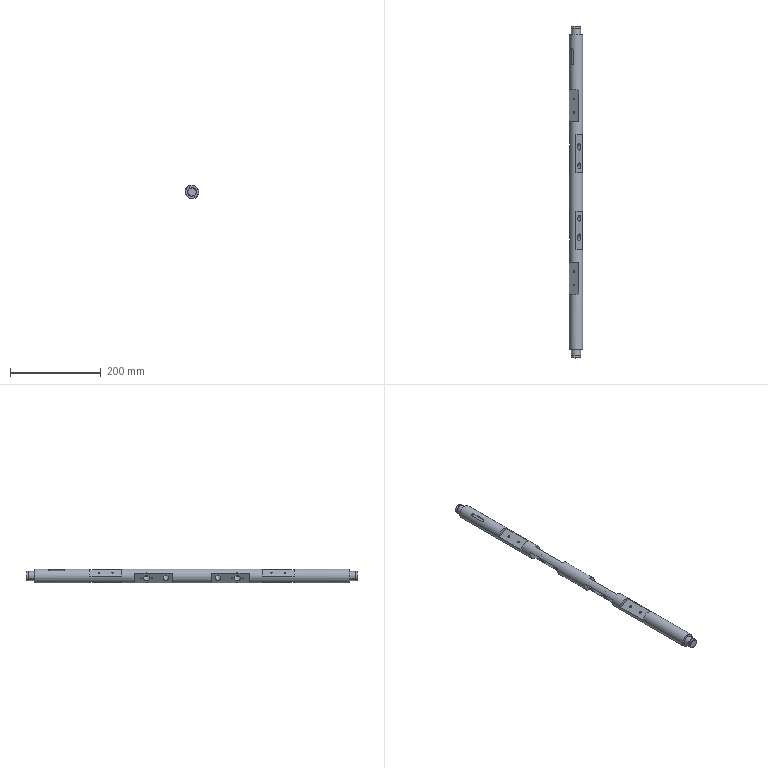Component | SolidWorks | SwingAxis1-1 | 1 solid | 116 faces | box 30 x 732 x 30 mm | volume 413852 mm3 | cylinder 49 | plane 35 | cone 32 | commonest cylinder face diameters 2.5 x16 4.2 x8 20 x8 15 x4 19 x4 12.5 x4 6 x3 30 x2 | material 45
build123d program:
from build123d import *

# Parameters (mm, degrees)
SKETCH1_R               = 15
BOSS_EXTRUDE1_DEPTH     = 696
SKETCH2_R               = 10
BOSS_EXTRUDE2_DEPTH     = 18
BOSS_EXTRUDE3_START     = 18
SKETCH3_R               = 10
BOSS_EXTRUDE3_DEPTH     = 18
CHAMFER1_SIZE           = 1
CUT_EXTRUDE1_START      = 11.5
CUT_EXTRUDE1_DEPTH      = 11.5
CUT_EXTRUDE2_DEPTH      = 715.315
CUT_EXTRUDE2_DEPTH_BACK = 715.315
SKETCH6_R               = 6.25
CUT_EXTRUDE3_DEPTH      = 715.528
SKETCH7_W               = 1
SKETCH7_H               = 1.2
CHAMFER2_SIZE           = 0.3
SKETCH8_R               = 7.5
CUT_EXTRUDE4_DEPTH      = 715.528
M3_TAPPED_HOLE1_D       = 2.5
M3_TAPPED_HOLE1_DEPTH   = 7.5
M3_TAPPED_HOLE1_TIP     = 0.7511
CUT_EXTRUDE5_DEPTH      = 715.315
CUT_EXTRUDE5_DEPTH_BACK = 715.315
SKETCH14_W              = 70
SKETCH14_H              = 39.9
SKETCH14_H_2            = 23.419
SKETCH14_H_3            = 27.126
M5_TAPPED_HOLE1_D       = 4.2


with BuildPart() as part:
    # Sketch1 → Boss-Extrude1 (new body)
    with BuildSketch(Plane.XY):
        Circle(SKETCH1_R)
    extrude(amount=BOSS_EXTRUDE1_DEPTH)

    # Sketch2 → Boss-Extrude2 (add)
    with BuildSketch(Plane.XY.offset(696)):
        Circle(SKETCH2_R)
    extrude(amount=BOSS_EXTRUDE2_DEPTH)

    # Sketch3 → Boss-Extrude3 (add)
    with BuildSketch(Plane(origin=(0, 0, 0), x_dir=(-1, 0, 0), z_dir=(0, 0, -1)).offset(BOSS_EXTRUDE3_START)):
        with Locations(Location((0, 0, 0), (0, 0, 180))):
            Circle(SKETCH3_R)
    extrude(amount=-BOSS_EXTRUDE3_DEPTH)

    # Chamfer1
    chamfer1_edges = [part.edges().sort_by_distance(p)[0] for p in [
        (-10, 0, -18),
        (-15, 0, 0),
        (-15, 0, 696),
        (-10, 0, 714),
    ]]
    chamfer(chamfer1_edges, length=CHAMFER1_SIZE)

    # Sketch4 → Cut-Extrude1 (cut)
    with BuildSketch(Plane(origin=(0, 0, 0), x_dir=(1, 0, 0), z_dir=(0, 1, 0)).offset(CUT_EXTRUDE1_START)):
        with BuildLine():
            Line((-3, -65), (-3, -35))
            ThreePointArc((-3, -35), (0, -32), (3, -35))
            Line((3, -35), (3, -65))
            ThreePointArc((3, -65), (0, -68), (-3, -65))
        make_face()
    extrude(amount=CUT_EXTRUDE1_DEPTH, mode=Mode.SUBTRACT)

    # Sketch5 → Cut-Extrude2 (cut, two sides: drawn at the far end of the back side and taken through both)
    with BuildSketch(Plane(origin=(0, 0, 0), x_dir=(1, 0, 0), z_dir=(0, 1, 0)).offset(-CUT_EXTRUDE2_DEPTH_BACK)):
        Polygon((-28, -275.5), (-28, -305.5), (-8, -305.5), (-8, -275.5), (-8, -220.5), (-28.473, -220.5), (-28.473, -275.5), align=None)
        Polygon((28, -275.5), (28, -305.5), (8, -305.5), (8, -275.5), (8, -220.5), (28.473, -220.5), (28.473, -275.5), align=None)
        Polygon((-28, -390.5), (-8, -390.5), (-8, -420.5), (-8, -475.5), (-37.779, -475.5), (-37.779, -420.5), (-28, -420.5), align=None)
        Polygon((28, -390.5), (8, -390.5), (8, -420.5), (8, -475.5), (37.779, -475.5), (37.779, -420.5), (28, -420.5), align=None)
    extrude(amount=CUT_EXTRUDE2_DEPTH + CUT_EXTRUDE2_DEPTH_BACK, mode=Mode.SUBTRACT)

    # Sketch6 → Cut-Extrude3 (cut, through all)
    with BuildSketch(Plane.ZY.offset(8)):
        with Locations((405.5, 0)):
            Circle(SKETCH6_R)
        with Locations((290.5, 0)):
            Circle(SKETCH6_R)
    extrude(amount=-CUT_EXTRUDE3_DEPTH, mode=Mode.SUBTRACT)

    # Sketch7 → Cut-Revolve1 (revolve, cut)
    with BuildSketch(Plane(origin=(0, 0, 0), x_dir=(1, 0, 0), z_dir=(0, 1, 0))):
        with Locations((-10, 12.6)):
            Rectangle(SKETCH7_W, SKETCH7_H)
        with Locations((-10, -708.6)):
            Rectangle(SKETCH7_W, SKETCH7_H)
    revolve(axis=Axis((0, 0, -18), (0, 0, 1)), mode=Mode.SUBTRACT)

    # Chamfer2
    chamfer2_edges = [part.edges().sort_by_distance(p)[0] for p in [
        (8, 0, 399.25),
        (-8, 0, 399.25),
        (8, 0, 284.25),
        (-8, 0, 284.25),
    ]]
    chamfer(chamfer2_edges, length=CHAMFER2_SIZE)

    # Sketch8 → Cut-Extrude4 (cut, through all)
    with BuildSketch(Plane.ZY.offset(8)):
        with Locations((248, 0)):
            Circle(SKETCH8_R)
        with Locations((448, 0)):
            Circle(SKETCH8_R)
    extrude(amount=-CUT_EXTRUDE4_DEPTH, mode=Mode.SUBTRACT)

    # M3 Tapped Hole1
    with Locations(Plane.ZY.offset(8)):
        with Locations((236, 0), (260, 0), (248, 12), (248, -12), (436, 0), (460, 0), (448, 12), (448, -12)):
            Hole(M3_TAPPED_HOLE1_D / 2, depth=M3_TAPPED_HOLE1_DEPTH)
            with Locations((0, 0, -(M3_TAPPED_HOLE1_DEPTH + M3_TAPPED_HOLE1_TIP / 2))):  # 118° drill point
                Cone(0, M3_TAPPED_HOLE1_D / 2, M3_TAPPED_HOLE1_TIP, mode=Mode.SUBTRACT)

    # Sketch14 → Cut-Extrude5 (cut, two sides: drawn at the far end of the back side and taken through both)
    with BuildSketch(Plane(origin=(0, 0, 0), x_dir=(0, 0, -1), z_dir=(1, 0, 0)).offset(-CUT_EXTRUDE5_DEPTH_BACK)):
        with Locations((-158, -27.95)):
            Rectangle(SKETCH14_W, SKETCH14_H)
        with Locations((-538, -27.95)):
            Rectangle(SKETCH14_W, SKETCH14_H)
        with Locations((-538, 19.71)):
            Rectangle(SKETCH14_W, SKETCH14_H_2)
        with Locations((-158, 21.563)):
            Rectangle(SKETCH14_W, SKETCH14_H_3)
    extrude(amount=CUT_EXTRUDE5_DEPTH + CUT_EXTRUDE5_DEPTH_BACK, mode=Mode.SUBTRACT)

    # M5 Tapped Hole1 (through all)
    with Locations(Plane(origin=(0, -8, 0), x_dir=(-1, 0, 0), z_dir=(0, -1, 0))):
        with Locations((0, -553), (0, -523), (0, -173), (0, -143)):
            Hole(M5_TAPPED_HOLE1_D / 2)


solid = part.part

# Placed as in the assembly
solid = solid.moved(Location((-28.685, 307.546, 10.43), (90, 0, 33.165)))